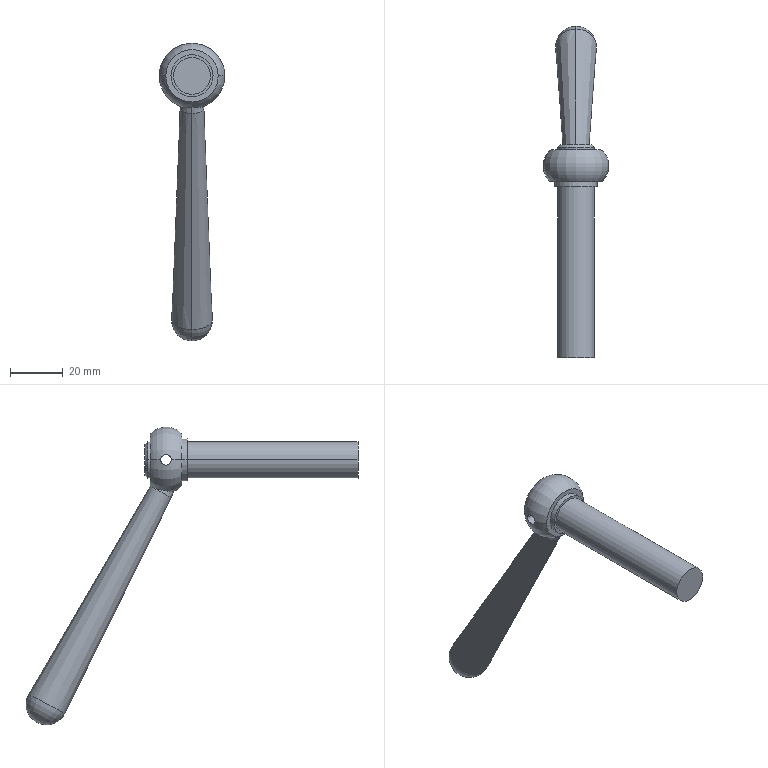Component | SolidWorks | Handle-1 | 1 solid | 23 faces | volume 27831 mm3 | cylinder 8 | cone 6 | plane 5 | torus 4 | commonest cylinder face diameters 14 x4 4 x2 16 x2
STEP:
#1=CARTESIAN_POINT('',(-2.717,8.526,-2.461));
#2=VERTEX_POINT('',#1);
#3=CARTESIAN_POINT('',(-3.189,8.526,-2.461));
#4=VERTEX_POINT('',#3);
#5=CARTESIAN_POINT('',(-2.953,8.526,-2.461));
#6=DIRECTION('',(0.,1.,0.));
#7=DIRECTION('',(1.,0.,0.));
#8=AXIS2_PLACEMENT_3D('',#5,#6,#7);
#9=CIRCLE('',#8,0.2362);
#10=EDGE_CURVE('',#2,#4,#9,.T.);
#11=ORIENTED_EDGE('',*,*,#10,.F.);
#12=CARTESIAN_POINT('',(-2.677,8.487,-2.461));
#13=VERTEX_POINT('',#12);
#14=CARTESIAN_POINT('',(-2.717,8.526,-2.461));
#15=DIRECTION('',(0.7071,-0.7071,-0.));
#16=VECTOR('',#15,39.37);
#17=LINE('',#14,#16);
#18=EDGE_CURVE('',#2,#13,#17,.T.);
#19=ORIENTED_EDGE('',*,*,#18,.T.);
#20=CARTESIAN_POINT('',(-3.228,8.487,-2.461));
#21=VERTEX_POINT('',#20);
#22=CARTESIAN_POINT('',(-2.953,8.487,-2.461));
#23=DIRECTION('',(0.,-1.,0.));
#24=DIRECTION('',(1.,0.,0.));
#25=AXIS2_PLACEMENT_3D('',#22,#23,#24);
#26=CIRCLE('',#25,0.2756);
#27=EDGE_CURVE('',#21,#13,#26,.T.);
#28=ORIENTED_EDGE('',*,*,#27,.F.);
#29=CARTESIAN_POINT('',(-3.189,8.526,-2.461));
#30=DIRECTION('',(-0.7071,-0.7071,0.));
#31=VECTOR('',#30,39.37);
#32=LINE('',#29,#31);
#33=EDGE_CURVE('',#4,#21,#32,.T.);
#34=ORIENTED_EDGE('',*,*,#33,.F.);
#35=EDGE_LOOP('',(#11,#19,#28,#34));
#36=FACE_OUTER_BOUND('',#35,.T.);
#37=CARTESIAN_POINT('',(-2.953,8.526,-2.461));
#38=DIRECTION('',(0.,-1.,0.));
#39=DIRECTION('',(-1.,0.,0.));
#40=AXIS2_PLACEMENT_3D('',#37,#38,#39);
#41=CONICAL_SURFACE('',#40,0.2362,0.7854);
#42=ADVANCED_FACE('',(#36),#41,.T.);
#43=ORIENTED_EDGE('',*,*,#27,.T.);
#44=CARTESIAN_POINT('',(-2.677,8.447,-2.461));
#45=VERTEX_POINT('',#44);
#46=CARTESIAN_POINT('',(-2.677,8.526,-2.461));
#47=DIRECTION('',(0.,-1.,0.));
#48=VECTOR('',#47,39.37);
#49=LINE('',#46,#48);
#50=EDGE_CURVE('',#13,#45,#49,.T.);
#51=ORIENTED_EDGE('',*,*,#50,.T.);
#52=CARTESIAN_POINT('',(-3.228,8.447,-2.461));
#53=VERTEX_POINT('',#52);
#54=CARTESIAN_POINT('',(-2.953,8.447,-2.461));
#55=DIRECTION('',(0.,1.,0.));
#56=DIRECTION('',(1.,0.,0.));
#57=AXIS2_PLACEMENT_3D('',#54,#55,#56);
#58=CIRCLE('',#57,0.2756);
#59=EDGE_CURVE('',#45,#53,#58,.T.);
#60=ORIENTED_EDGE('',*,*,#59,.T.);
#61=CARTESIAN_POINT('',(-3.228,8.526,-2.461));
#62=DIRECTION('',(0.,-1.,0.));
#63=VECTOR('',#62,39.37);
#64=LINE('',#61,#63);
#65=EDGE_CURVE('',#21,#53,#64,.T.);
#66=ORIENTED_EDGE('',*,*,#65,.F.);
#67=EDGE_LOOP('',(#43,#51,#60,#66));
#68=FACE_OUTER_BOUND('',#67,.T.);
#69=CARTESIAN_POINT('',(-2.953,8.526,-2.461));
#70=DIRECTION('',(0.,-1.,0.));
#71=DIRECTION('',(-1.,0.,0.));
#72=AXIS2_PLACEMENT_3D('',#69,#70,#71);
#73=CYLINDRICAL_SURFACE('',#72,0.2756);
#74=ADVANCED_FACE('',(#68),#73,.T.);
#75=CARTESIAN_POINT('',(-3.434,8.29,-2.461));
#76=VERTEX_POINT('',#75);
#77=CARTESIAN_POINT('',(-3.434,8.132,-2.461));
#78=VERTEX_POINT('',#77);
#79=CARTESIAN_POINT('',(-3.434,8.29,-2.461));
#80=CARTESIAN_POINT('',(-3.434,8.29,-2.455));
#81=CARTESIAN_POINT('',(-3.434,8.289,-2.45));
#82=CARTESIAN_POINT('',(-3.434,8.287,-2.44));
#83=CARTESIAN_POINT('',(-3.434,8.286,-2.435));
#84=CARTESIAN_POINT('',(-3.434,8.282,-2.426));
#85=CARTESIAN_POINT('',(-3.435,8.28,-2.421));
#86=CARTESIAN_POINT('',(-3.435,8.274,-2.413));
#87=CARTESIAN_POINT('',(-3.435,8.271,-2.409));
#88=CARTESIAN_POINT('',(-3.436,8.26,-2.398));
#89=CARTESIAN_POINT('',(-3.436,8.251,-2.392));
#90=CARTESIAN_POINT('',(-3.437,8.237,-2.386));
#91=CARTESIAN_POINT('',(-3.437,8.232,-2.384));
#92=CARTESIAN_POINT('',(-3.437,8.222,-2.382));
#93=CARTESIAN_POINT('',(-3.437,8.216,-2.382));
#94=CARTESIAN_POINT('',(-3.437,8.206,-2.382));
#95=CARTESIAN_POINT('',(-3.437,8.201,-2.382));
#96=CARTESIAN_POINT('',(-3.437,8.191,-2.384));
#97=CARTESIAN_POINT('',(-3.437,8.186,-2.386));
#98=CARTESIAN_POINT('',(-3.436,8.172,-2.392));
#99=CARTESIAN_POINT('',(-3.436,8.163,-2.398));
#100=CARTESIAN_POINT('',(-3.435,8.152,-2.409));
#101=CARTESIAN_POINT('',(-3.435,8.149,-2.413));
#102=CARTESIAN_POINT('',(-3.435,8.143,-2.421));
#103=CARTESIAN_POINT('',(-3.434,8.14,-2.426));
#104=CARTESIAN_POINT('',(-3.434,8.136,-2.435));
#105=CARTESIAN_POINT('',(-3.434,8.135,-2.44));
#106=CARTESIAN_POINT('',(-3.434,8.133,-2.45));
#107=CARTESIAN_POINT('',(-3.434,8.132,-2.455));
#108=CARTESIAN_POINT('',(-3.434,8.132,-2.461));
#109=B_SPLINE_CURVE_WITH_KNOTS('',3,(#79,#80,#81,#82,#83,#84,#85,#86,#87,#88,#89,#90,#91,#92,#93,#94,#95,#96,#97,#98,#99,#100,#101,#102,#103,#104,#105,#106,#107,#108),.UNSPECIFIED.,.F.,.F.,(4,2,2,2,2,2,2,2,2,2,2,2,2,2,4),(0.007793,0.008184,0.008575,0.008965,0.009356,0.01014,0.01053,0.01092,0.01131,0.0117,0.01248,0.01287,0.01326,0.01365,0.01405),.UNSPECIFIED.);
#110=EDGE_CURVE('',#76,#78,#109,.T.);
#111=ORIENTED_EDGE('',*,*,#110,.F.);
#112=CARTESIAN_POINT('',(-2.472,8.29,-2.461));
#113=VERTEX_POINT('',#112);
#114=CARTESIAN_POINT('',(-3.613,8.29,-2.461));
#115=DIRECTION('',(1.,0.,0.));
#116=VECTOR('',#115,39.37);
#117=LINE('',#114,#116);
#118=EDGE_CURVE('',#76,#113,#117,.T.);
#119=ORIENTED_EDGE('',*,*,#118,.T.);
#120=CARTESIAN_POINT('',(-2.472,8.132,-2.461));
#121=VERTEX_POINT('',#120);
#122=CARTESIAN_POINT('',(-2.472,8.132,-2.461));
#123=CARTESIAN_POINT('',(-2.472,8.132,-2.45));
#124=CARTESIAN_POINT('',(-2.471,8.135,-2.44));
#125=CARTESIAN_POINT('',(-2.471,8.142,-2.421));
#126=CARTESIAN_POINT('',(-2.471,8.148,-2.412));
#127=CARTESIAN_POINT('',(-2.47,8.159,-2.401));
#128=CARTESIAN_POINT('',(-2.47,8.163,-2.398));
#129=CARTESIAN_POINT('',(-2.469,8.172,-2.392));
#130=CARTESIAN_POINT('',(-2.469,8.176,-2.39));
#131=CARTESIAN_POINT('',(-2.469,8.186,-2.386));
#132=CARTESIAN_POINT('',(-2.469,8.191,-2.384));
#133=CARTESIAN_POINT('',(-2.469,8.201,-2.382));
#134=CARTESIAN_POINT('',(-2.469,8.206,-2.382));
#135=CARTESIAN_POINT('',(-2.469,8.222,-2.382));
#136=CARTESIAN_POINT('',(-2.469,8.232,-2.384));
#137=CARTESIAN_POINT('',(-2.469,8.246,-2.39));
#138=CARTESIAN_POINT('',(-2.469,8.251,-2.392));
#139=CARTESIAN_POINT('',(-2.47,8.259,-2.398));
#140=CARTESIAN_POINT('',(-2.47,8.263,-2.401));
#141=CARTESIAN_POINT('',(-2.47,8.271,-2.409));
#142=CARTESIAN_POINT('',(-2.471,8.274,-2.413));
#143=CARTESIAN_POINT('',(-2.471,8.28,-2.421));
#144=CARTESIAN_POINT('',(-2.471,8.282,-2.426));
#145=CARTESIAN_POINT('',(-2.471,8.286,-2.435));
#146=CARTESIAN_POINT('',(-2.471,8.287,-2.44));
#147=CARTESIAN_POINT('',(-2.472,8.289,-2.45));
#148=CARTESIAN_POINT('',(-2.472,8.29,-2.455));
#149=CARTESIAN_POINT('',(-2.472,8.29,-2.461));
#150=B_SPLINE_CURVE_WITH_KNOTS('',3,(#122,#123,#124,#125,#126,#127,#128,#129,#130,#131,#132,#133,#134,#135,#136,#137,#138,#139,#140,#141,#142,#143,#144,#145,#146,#147,#148,#149),.UNSPECIFIED.,.F.,.F.,(4,2,2,2,2,2,2,2,2,2,2,2,2,4),(0.01097,0.01176,0.01254,0.01293,0.01332,0.01371,0.0141,0.01488,0.01527,0.01566,0.01606,0.01645,0.01684,0.01723),.UNSPECIFIED.);
#151=EDGE_CURVE('',#121,#113,#150,.T.);
#152=ORIENTED_EDGE('',*,*,#151,.F.);
#153=CARTESIAN_POINT('',(-3.613,8.132,-2.461));
#154=DIRECTION('',(1.,0.,0.));
#155=VECTOR('',#154,39.37);
#156=LINE('',#153,#155);
#157=EDGE_CURVE('',#78,#121,#156,.T.);
#158=ORIENTED_EDGE('',*,*,#157,.F.);
#159=EDGE_LOOP('',(#111,#119,#152,#158));
#160=FACE_OUTER_BOUND('',#159,.T.);
#161=CARTESIAN_POINT('',(-3.613,8.211,-2.461));
#162=DIRECTION('',(1.,0.,0.));
#163=DIRECTION('',(0.,-1.,0.));
#164=AXIS2_PLACEMENT_3D('',#161,#162,#163);
#165=CYLINDRICAL_SURFACE('',#164,0.07874);
#166=ADVANCED_FACE('',(#160),#165,.F.);
#167=CARTESIAN_POINT('',(-2.953,10.146,-6.391));
#168=VERTEX_POINT('',#167);
#169=CARTESIAN_POINT('',(-2.953,9.726,-6.258));
#170=VERTEX_POINT('',#169);
#171=CARTESIAN_POINT('',(-2.953,10.,-6.123));
#172=DIRECTION('',(-1.,0.,0.));
#173=DIRECTION('',(0.,0.,1.));
#174=AXIS2_PLACEMENT_3D('',#171,#172,#173);
#175=CIRCLE('',#174,0.305);
#176=EDGE_CURVE('',#168,#170,#175,.T.);
#177=ORIENTED_EDGE('',*,*,#176,.F.);
#178=CARTESIAN_POINT('',(-2.953,10.266,-5.967));
#179=VERTEX_POINT('',#178);
#180=CARTESIAN_POINT('',(-2.953,10.003,-6.121));
#181=DIRECTION('',(1.,-0.,-0.));
#182=DIRECTION('',(0.,1.,0.));
#183=AXIS2_PLACEMENT_3D('',#180,#181,#182);
#184=CIRCLE('',#183,0.305);
#185=EDGE_CURVE('',#168,#179,#184,.T.);
#186=ORIENTED_EDGE('',*,*,#185,.T.);
#187=CARTESIAN_POINT('',(-2.953,9.996,-6.113));
#188=DIRECTION('',(0.,-0.4737,0.8807));
#189=DIRECTION('',(0.,-0.8807,-0.4737));
#190=AXIS2_PLACEMENT_3D('',#187,#188,#189);
#191=CIRCLE('',#190,0.3066);
#192=EDGE_CURVE('',#170,#179,#191,.T.);
#193=ORIENTED_EDGE('',*,*,#192,.F.);
#194=EDGE_LOOP('',(#177,#186,#193));
#195=FACE_OUTER_BOUND('',#194,.T.);
#196=CARTESIAN_POINT('',(-2.953,10.002,-6.122));
#197=DIRECTION('',(0.,-0.4737,0.8807));
#198=DIRECTION('',(0.,-0.8807,-0.4737));
#199=AXIS2_PLACEMENT_3D('',#196,#197,#198);
#200=TOROIDAL_SURFACE('',#199,0.001727,0.305);
#201=ADVANCED_FACE('',(#195),#200,.T.);
#202=CARTESIAN_POINT('',(-2.953,8.131,-3.023));
#203=VERTEX_POINT('',#202);
#204=CARTESIAN_POINT('',(-2.953,8.447,-2.853));
#205=VERTEX_POINT('',#204);
#206=CARTESIAN_POINT('',(-2.953,8.289,-2.938));
#207=DIRECTION('',(0.,-0.4737,0.8807));
#208=DIRECTION('',(0.,-0.8807,-0.4737));
#209=AXIS2_PLACEMENT_3D('',#206,#207,#208);
#210=CIRCLE('',#209,0.1796);
#211=EDGE_CURVE('',#203,#205,#210,.T.);
#212=ORIENTED_EDGE('',*,*,#211,.F.);
#213=CARTESIAN_POINT('',(-2.953,9.726,-6.258));
#214=DIRECTION('',(0.,0.4423,-0.8968));
#215=VECTOR('',#214,39.37);
#216=LINE('',#213,#215);
#217=EDGE_CURVE('',#203,#170,#216,.T.);
#218=ORIENTED_EDGE('',*,*,#217,.T.);
#219=ORIENTED_EDGE('',*,*,#192,.T.);
#220=CARTESIAN_POINT('',(-2.953,10.266,-5.967));
#221=DIRECTION('',(0.,0.5044,-0.8635));
#222=VECTOR('',#221,39.37);
#223=LINE('',#220,#222);
#224=EDGE_CURVE('',#205,#179,#223,.T.);
#225=ORIENTED_EDGE('',*,*,#224,.F.);
#226=EDGE_LOOP('',(#212,#218,#219,#225));
#227=FACE_OUTER_BOUND('',#226,.T.);
#228=CARTESIAN_POINT('',(-2.953,9.996,-6.113));
#229=DIRECTION('',(0.,0.4737,-0.8807));
#230=DIRECTION('',(0.,0.8807,0.4737));
#231=AXIS2_PLACEMENT_3D('',#228,#229,#230);
#232=CONICAL_SURFACE('',#231,0.3066,0.03523);
#233=ADVANCED_FACE('',(#227),#232,.T.);
#234=CARTESIAN_POINT('',(-2.953,8.099,-2.932));
#235=VERTEX_POINT('',#234);
#236=CARTESIAN_POINT('',(-2.953,8.099,-2.932));
#237=CARTESIAN_POINT('',(-2.941,8.099,-2.932));
#238=CARTESIAN_POINT('',(-2.93,8.1,-2.932));
#239=CARTESIAN_POINT('',(-2.907,8.106,-2.932));
#240=CARTESIAN_POINT('',(-2.896,8.109,-2.932));
#241=CARTESIAN_POINT('',(-2.875,8.119,-2.932));
#242=CARTESIAN_POINT('',(-2.865,8.125,-2.932));
#243=CARTESIAN_POINT('',(-2.846,8.139,-2.931));
#244=CARTESIAN_POINT('',(-2.837,8.146,-2.931));
#245=CARTESIAN_POINT('',(-2.821,8.163,-2.93));
#246=CARTESIAN_POINT('',(-2.814,8.173,-2.929));
#247=CARTESIAN_POINT('',(-2.802,8.192,-2.927));
#248=CARTESIAN_POINT('',(-2.796,8.202,-2.926));
#249=CARTESIAN_POINT('',(-2.788,8.224,-2.922));
#250=CARTESIAN_POINT('',(-2.784,8.235,-2.921));
#251=CARTESIAN_POINT('',(-2.779,8.257,-2.916));
#252=CARTESIAN_POINT('',(-2.778,8.268,-2.914));
#253=CARTESIAN_POINT('',(-2.778,8.291,-2.909));
#254=CARTESIAN_POINT('',(-2.778,8.302,-2.906));
#255=CARTESIAN_POINT('',(-2.782,8.324,-2.9));
#256=CARTESIAN_POINT('',(-2.786,8.335,-2.897));
#257=CARTESIAN_POINT('',(-2.794,8.355,-2.89));
#258=CARTESIAN_POINT('',(-2.799,8.365,-2.887));
#259=CARTESIAN_POINT('',(-2.812,8.384,-2.88));
#260=CARTESIAN_POINT('',(-2.819,8.392,-2.877));
#261=CARTESIAN_POINT('',(-2.836,8.408,-2.871));
#262=CARTESIAN_POINT('',(-2.845,8.414,-2.868));
#263=CARTESIAN_POINT('',(-2.864,8.426,-2.863));
#264=CARTESIAN_POINT('',(-2.874,8.431,-2.861));
#265=CARTESIAN_POINT('',(-2.896,8.439,-2.857));
#266=CARTESIAN_POINT('',(-2.907,8.442,-2.856));
#267=CARTESIAN_POINT('',(-2.93,8.446,-2.854));
#268=CARTESIAN_POINT('',(-2.941,8.447,-2.853));
#269=CARTESIAN_POINT('',(-2.953,8.447,-2.853));
#270=B_SPLINE_CURVE_WITH_KNOTS('',3,(#236,#237,#238,#239,#240,#241,#242,#243,#244,#245,#246,#247,#248,#249,#250,#251,#252,#253,#254,#255,#256,#257,#258,#259,#260,#261,#262,#263,#264,#265,#266,#267,#268,#269),.UNSPECIFIED.,.F.,.F.,(4,2,2,2,2,2,2,2,2,2,2,2,2,2,2,2,4),(0.003343,0.004223,0.005103,0.005984,0.006864,0.007744,0.008624,0.009504,0.01038,0.01126,0.01214,0.01302,0.0139,0.01478,0.01566,0.01654,0.01742),.UNSPECIFIED.);
#271=EDGE_CURVE('',#235,#205,#270,.T.);
#272=ORIENTED_EDGE('',*,*,#271,.F.);
#273=CARTESIAN_POINT('',(-2.953,8.131,-3.023));
#274=DIRECTION('',(0.,0.3301,-0.944));
#275=VECTOR('',#274,39.37);
#276=LINE('',#273,#275);
#277=EDGE_CURVE('',#235,#203,#276,.T.);
#278=ORIENTED_EDGE('',*,*,#277,.T.);
#279=ORIENTED_EDGE('',*,*,#211,.T.);
#280=EDGE_LOOP('',(#272,#278,#279));
#281=FACE_OUTER_BOUND('',#280,.T.);
#282=CARTESIAN_POINT('',(-2.953,8.289,-2.938));
#283=DIRECTION('',(0.,0.4737,-0.8807));
#284=DIRECTION('',(0.,0.8807,0.4737));
#285=AXIS2_PLACEMENT_3D('',#282,#283,#284);
#286=CONICAL_SURFACE('',#285,0.1796,0.1571);
#287=ADVANCED_FACE('',(#281),#286,.T.);
#288=CARTESIAN_POINT('',(-2.638,7.975,-2.461));
#289=VERTEX_POINT('',#288);
#290=CARTESIAN_POINT('',(-3.268,7.975,-2.461));
#291=VERTEX_POINT('',#290);
#292=CARTESIAN_POINT('',(-2.953,7.975,-2.461));
#293=DIRECTION('',(0.,1.,0.));
#294=DIRECTION('',(1.,0.,0.));
#295=AXIS2_PLACEMENT_3D('',#292,#293,#294);
#296=CIRCLE('',#295,0.315);
#297=EDGE_CURVE('',#289,#291,#296,.T.);
#298=ORIENTED_EDGE('',*,*,#297,.F.);
#299=CARTESIAN_POINT('',(-2.638,7.896,-2.461));
#300=VERTEX_POINT('',#299);
#301=CARTESIAN_POINT('',(-2.638,7.975,-2.461));
#302=DIRECTION('',(0.,-1.,0.));
#303=VECTOR('',#302,39.37);
#304=LINE('',#301,#303);
#305=EDGE_CURVE('',#289,#300,#304,.T.);
#306=ORIENTED_EDGE('',*,*,#305,.T.);
#307=CARTESIAN_POINT('',(-3.268,7.896,-2.461));
#308=VERTEX_POINT('',#307);
#309=CARTESIAN_POINT('',(-2.953,7.896,-2.461));
#310=DIRECTION('',(0.,1.,0.));
#311=DIRECTION('',(1.,0.,0.));
#312=AXIS2_PLACEMENT_3D('',#309,#310,#311);
#313=CIRCLE('',#312,0.315);
#314=EDGE_CURVE('',#300,#308,#313,.T.);
#315=ORIENTED_EDGE('',*,*,#314,.T.);
#316=CARTESIAN_POINT('',(-3.268,7.975,-2.461));
#317=DIRECTION('',(0.,-1.,0.));
#318=VECTOR('',#317,39.37);
#319=LINE('',#316,#318);
#320=EDGE_CURVE('',#291,#308,#319,.T.);
#321=ORIENTED_EDGE('',*,*,#320,.F.);
#322=EDGE_LOOP('',(#298,#306,#315,#321));
#323=FACE_OUTER_BOUND('',#322,.T.);
#324=CARTESIAN_POINT('',(-2.953,7.975,-2.461));
#325=DIRECTION('',(0.,-1.,0.));
#326=DIRECTION('',(-1.,0.,0.));
#327=AXIS2_PLACEMENT_3D('',#324,#325,#326);
#328=CYLINDRICAL_SURFACE('',#327,0.315);
#329=ADVANCED_FACE('',(#323),#328,.T.);
#330=CARTESIAN_POINT('',(-2.677,5.337,-2.461));
#331=VERTEX_POINT('',#330);
#332=CARTESIAN_POINT('',(-3.228,5.337,-2.461));
#333=VERTEX_POINT('',#332);
#334=CARTESIAN_POINT('',(-2.953,5.337,-2.461));
#335=DIRECTION('',(0.,1.,0.));
#336=DIRECTION('',(1.,0.,0.));
#337=AXIS2_PLACEMENT_3D('',#334,#335,#336);
#338=CIRCLE('',#337,0.2756);
#339=EDGE_CURVE('',#331,#333,#338,.T.);
#340=ORIENTED_EDGE('',*,*,#339,.T.);
#341=CARTESIAN_POINT('',(-3.228,7.896,-2.461));
#342=VERTEX_POINT('',#341);
#343=CARTESIAN_POINT('',(-3.228,5.337,-2.461));
#344=DIRECTION('',(0.,1.,0.));
#345=VECTOR('',#344,39.37);
#346=LINE('',#343,#345);
#347=EDGE_CURVE('',#333,#342,#346,.T.);
#348=ORIENTED_EDGE('',*,*,#347,.T.);
#349=CARTESIAN_POINT('',(-2.677,7.896,-2.461));
#350=VERTEX_POINT('',#349);
#351=CARTESIAN_POINT('',(-2.953,7.896,-2.461));
#352=DIRECTION('',(0.,1.,0.));
#353=DIRECTION('',(1.,0.,0.));
#354=AXIS2_PLACEMENT_3D('',#351,#352,#353);
#355=CIRCLE('',#354,0.2756);
#356=EDGE_CURVE('',#350,#342,#355,.T.);
#357=ORIENTED_EDGE('',*,*,#356,.F.);
#358=CARTESIAN_POINT('',(-2.677,5.337,-2.461));
#359=DIRECTION('',(0.,1.,0.));
#360=VECTOR('',#359,39.37);
#361=LINE('',#358,#360);
#362=EDGE_CURVE('',#331,#350,#361,.T.);
#363=ORIENTED_EDGE('',*,*,#362,.F.);
#364=EDGE_LOOP('',(#340,#348,#357,#363));
#365=FACE_OUTER_BOUND('',#364,.T.);
#366=CARTESIAN_POINT('',(-2.953,5.337,-2.461));
#367=DIRECTION('',(0.,1.,0.));
#368=DIRECTION('',(1.,0.,0.));
#369=AXIS2_PLACEMENT_3D('',#366,#367,#368);
#370=CYLINDRICAL_SURFACE('',#369,0.2756);
#371=ADVANCED_FACE('',(#365),#370,.T.);
#372=CARTESIAN_POINT('',(-2.56,7.975,-2.461));
#373=VERTEX_POINT('',#372);
#374=CARTESIAN_POINT('',(-3.345,7.975,-2.461));
#375=VERTEX_POINT('',#374);
#376=CARTESIAN_POINT('',(-2.953,7.975,-2.461));
#377=DIRECTION('',(0.,1.,0.));
#378=DIRECTION('',(1.,0.,0.));
#379=AXIS2_PLACEMENT_3D('',#376,#377,#378);
#380=CIRCLE('',#379,0.3927);
#381=EDGE_CURVE('',#373,#375,#380,.T.);
#382=ORIENTED_EDGE('',*,*,#381,.T.);
#383=CARTESIAN_POINT('',(-3.109,8.211,-2.461));
#384=DIRECTION('',(0.,0.,-1.));
#385=DIRECTION('',(-1.,0.,0.));
#386=AXIS2_PLACEMENT_3D('',#383,#384,#385);
#387=CIRCLE('',#386,0.3341);
#388=EDGE_CURVE('',#375,#78,#387,.T.);
#389=ORIENTED_EDGE('',*,*,#388,.T.);
#390=CARTESIAN_POINT('',(-3.434,8.132,-2.461));
#391=CARTESIAN_POINT('',(-3.434,8.132,-2.466));
#392=CARTESIAN_POINT('',(-3.434,8.133,-2.471));
#393=CARTESIAN_POINT('',(-3.434,8.135,-2.481));
#394=CARTESIAN_POINT('',(-3.434,8.136,-2.486));
#395=CARTESIAN_POINT('',(-3.435,8.142,-2.5));
#396=CARTESIAN_POINT('',(-3.435,8.148,-2.509));
#397=CARTESIAN_POINT('',(-3.436,8.159,-2.52));
#398=CARTESIAN_POINT('',(-3.436,8.163,-2.523));
#399=CARTESIAN_POINT('',(-3.436,8.172,-2.529));
#400=CARTESIAN_POINT('',(-3.436,8.176,-2.531));
#401=CARTESIAN_POINT('',(-3.437,8.186,-2.535));
#402=CARTESIAN_POINT('',(-3.437,8.191,-2.537));
#403=CARTESIAN_POINT('',(-3.437,8.201,-2.539));
#404=CARTESIAN_POINT('',(-3.437,8.206,-2.539));
#405=CARTESIAN_POINT('',(-3.437,8.222,-2.539));
#406=CARTESIAN_POINT('',(-3.437,8.232,-2.537));
#407=CARTESIAN_POINT('',(-3.436,8.246,-2.531));
#408=CARTESIAN_POINT('',(-3.436,8.251,-2.529));
#409=CARTESIAN_POINT('',(-3.436,8.259,-2.523));
#410=CARTESIAN_POINT('',(-3.436,8.263,-2.52));
#411=CARTESIAN_POINT('',(-3.435,8.271,-2.513));
#412=CARTESIAN_POINT('',(-3.435,8.274,-2.509));
#413=CARTESIAN_POINT('',(-3.435,8.28,-2.5));
#414=CARTESIAN_POINT('',(-3.434,8.282,-2.495));
#415=CARTESIAN_POINT('',(-3.434,8.288,-2.481));
#416=CARTESIAN_POINT('',(-3.434,8.29,-2.471));
#417=CARTESIAN_POINT('',(-3.434,8.29,-2.461));
#418=B_SPLINE_CURVE_WITH_KNOTS('',3,(#390,#391,#392,#393,#394,#395,#396,#397,#398,#399,#400,#401,#402,#403,#404,#405,#406,#407,#408,#409,#410,#411,#412,#413,#414,#415,#416,#417),.UNSPECIFIED.,.F.,.F.,(4,2,2,2,2,2,2,2,2,2,2,2,2,4),(0.001536,0.001927,0.002318,0.003101,0.003492,0.003883,0.004274,0.004665,0.005447,0.005838,0.006229,0.00662,0.007011,0.007793),.UNSPECIFIED.);
#419=EDGE_CURVE('',#78,#76,#418,.T.);
#420=ORIENTED_EDGE('',*,*,#419,.T.);
#421=CARTESIAN_POINT('',(-3.345,8.447,-2.461));
#422=VERTEX_POINT('',#421);
#423=CARTESIAN_POINT('',(-3.109,8.211,-2.461));
#424=DIRECTION('',(0.,0.,-1.));
#425=DIRECTION('',(-1.,0.,0.));
#426=AXIS2_PLACEMENT_3D('',#423,#424,#425);
#427=CIRCLE('',#426,0.3341);
#428=EDGE_CURVE('',#76,#422,#427,.T.);
#429=ORIENTED_EDGE('',*,*,#428,.T.);
#430=CARTESIAN_POINT('',(-2.953,8.447,-2.461));
#431=DIRECTION('',(0.,1.,0.));
#432=DIRECTION('',(1.,0.,0.));
#433=AXIS2_PLACEMENT_3D('',#430,#431,#432);
#434=CIRCLE('',#433,0.3927);
#435=EDGE_CURVE('',#205,#422,#434,.T.);
#436=ORIENTED_EDGE('',*,*,#435,.F.);
#437=CARTESIAN_POINT('',(-2.953,8.447,-2.853));
#438=CARTESIAN_POINT('',(-2.964,8.447,-2.853));
#439=CARTESIAN_POINT('',(-2.976,8.446,-2.854));
#440=CARTESIAN_POINT('',(-2.999,8.442,-2.856));
#441=CARTESIAN_POINT('',(-3.01,8.439,-2.857));
#442=CARTESIAN_POINT('',(-3.031,8.431,-2.861));
#443=CARTESIAN_POINT('',(-3.042,8.426,-2.863));
#444=CARTESIAN_POINT('',(-3.061,8.414,-2.868));
#445=CARTESIAN_POINT('',(-3.07,8.408,-2.871));
#446=CARTESIAN_POINT('',(-3.086,8.392,-2.877));
#447=CARTESIAN_POINT('',(-3.093,8.384,-2.88));
#448=CARTESIAN_POINT('',(-3.106,8.365,-2.887));
#449=CARTESIAN_POINT('',(-3.111,8.355,-2.89));
#450=CARTESIAN_POINT('',(-3.12,8.335,-2.897));
#451=CARTESIAN_POINT('',(-3.123,8.324,-2.9));
#452=CARTESIAN_POINT('',(-3.127,8.302,-2.906));
#453=CARTESIAN_POINT('',(-3.128,8.291,-2.909));
#454=CARTESIAN_POINT('',(-3.128,8.268,-2.914));
#455=CARTESIAN_POINT('',(-3.126,8.257,-2.916));
#456=CARTESIAN_POINT('',(-3.121,8.234,-2.921));
#457=CARTESIAN_POINT('',(-3.118,8.223,-2.922));
#458=CARTESIAN_POINT('',(-3.109,8.202,-2.926));
#459=CARTESIAN_POINT('',(-3.104,8.192,-2.927));
#460=CARTESIAN_POINT('',(-3.091,8.172,-2.929));
#461=CARTESIAN_POINT('',(-3.084,8.163,-2.93));
#462=CARTESIAN_POINT('',(-3.068,8.146,-2.931));
#463=CARTESIAN_POINT('',(-3.059,8.139,-2.931));
#464=CARTESIAN_POINT('',(-3.041,8.125,-2.932));
#465=CARTESIAN_POINT('',(-3.031,8.119,-2.932));
#466=CARTESIAN_POINT('',(-3.01,8.109,-2.932));
#467=CARTESIAN_POINT('',(-2.999,8.106,-2.932));
#468=CARTESIAN_POINT('',(-2.976,8.1,-2.932));
#469=CARTESIAN_POINT('',(-2.964,8.099,-2.932));
#470=CARTESIAN_POINT('',(-2.953,8.099,-2.932));
#471=B_SPLINE_CURVE_WITH_KNOTS('',3,(#437,#438,#439,#440,#441,#442,#443,#444,#445,#446,#447,#448,#449,#450,#451,#452,#453,#454,#455,#456,#457,#458,#459,#460,#461,#462,#463,#464,#465,#466,#467,#468,#469,#470),.UNSPECIFIED.,.F.,.F.,(4,2,2,2,2,2,2,2,2,2,2,2,2,2,2,2,4),(0.01742,0.0183,0.01918,0.02006,0.02094,0.02182,0.0227,0.02358,0.02446,0.02534,0.02622,0.0271,0.02798,0.02886,0.02974,0.03062,0.0315),.UNSPECIFIED.);
#472=EDGE_CURVE('',#205,#235,#471,.T.);
#473=ORIENTED_EDGE('',*,*,#472,.T.);
#474=ORIENTED_EDGE('',*,*,#271,.T.);
#475=CARTESIAN_POINT('',(-2.56,8.447,-2.461));
#476=VERTEX_POINT('',#475);
#477=CARTESIAN_POINT('',(-2.953,8.447,-2.461));
#478=DIRECTION('',(0.,1.,0.));
#479=DIRECTION('',(1.,0.,0.));
#480=AXIS2_PLACEMENT_3D('',#477,#478,#479);
#481=CIRCLE('',#480,0.3927);
#482=EDGE_CURVE('',#476,#205,#481,.T.);
#483=ORIENTED_EDGE('',*,*,#482,.F.);
#484=CARTESIAN_POINT('',(-2.796,8.211,-2.461));
#485=DIRECTION('',(0.,0.,1.));
#486=DIRECTION('',(1.,0.,0.));
#487=AXIS2_PLACEMENT_3D('',#484,#485,#486);
#488=CIRCLE('',#487,0.3341);
#489=EDGE_CURVE('',#113,#476,#488,.T.);
#490=ORIENTED_EDGE('',*,*,#489,.F.);
#491=CARTESIAN_POINT('',(-2.472,8.29,-2.461));
#492=CARTESIAN_POINT('',(-2.472,8.29,-2.466));
#493=CARTESIAN_POINT('',(-2.472,8.289,-2.471));
#494=CARTESIAN_POINT('',(-2.471,8.287,-2.481));
#495=CARTESIAN_POINT('',(-2.471,8.286,-2.486));
#496=CARTESIAN_POINT('',(-2.471,8.282,-2.496));
#497=CARTESIAN_POINT('',(-2.471,8.28,-2.5));
#498=CARTESIAN_POINT('',(-2.471,8.274,-2.509));
#499=CARTESIAN_POINT('',(-2.47,8.271,-2.513));
#500=CARTESIAN_POINT('',(-2.47,8.26,-2.524));
#501=CARTESIAN_POINT('',(-2.469,8.251,-2.529));
#502=CARTESIAN_POINT('',(-2.469,8.237,-2.535));
#503=CARTESIAN_POINT('',(-2.469,8.232,-2.537));
#504=CARTESIAN_POINT('',(-2.469,8.221,-2.539));
#505=CARTESIAN_POINT('',(-2.469,8.216,-2.539));
#506=CARTESIAN_POINT('',(-2.469,8.206,-2.539));
#507=CARTESIAN_POINT('',(-2.469,8.201,-2.539));
#508=CARTESIAN_POINT('',(-2.469,8.191,-2.537));
#509=CARTESIAN_POINT('',(-2.469,8.186,-2.535));
#510=CARTESIAN_POINT('',(-2.469,8.176,-2.531));
#511=CARTESIAN_POINT('',(-2.469,8.172,-2.529));
#512=CARTESIAN_POINT('',(-2.47,8.163,-2.523));
#513=CARTESIAN_POINT('',(-2.47,8.159,-2.52));
#514=CARTESIAN_POINT('',(-2.47,8.152,-2.513));
#515=CARTESIAN_POINT('',(-2.471,8.149,-2.509));
#516=CARTESIAN_POINT('',(-2.471,8.143,-2.5));
#517=CARTESIAN_POINT('',(-2.471,8.14,-2.496));
#518=CARTESIAN_POINT('',(-2.471,8.136,-2.486));
#519=CARTESIAN_POINT('',(-2.471,8.135,-2.481));
#520=CARTESIAN_POINT('',(-2.472,8.133,-2.471));
#521=CARTESIAN_POINT('',(-2.472,8.132,-2.466));
#522=CARTESIAN_POINT('',(-2.472,8.132,-2.461));
#523=B_SPLINE_CURVE_WITH_KNOTS('',3,(#491,#492,#493,#494,#495,#496,#497,#498,#499,#500,#501,#502,#503,#504,#505,#506,#507,#508,#509,#510,#511,#512,#513,#514,#515,#516,#517,#518,#519,#520,#521,#522),.UNSPECIFIED.,.F.,.F.,(4,2,2,2,2,2,2,2,2,2,2,2,2,2,2,4),(0.004719,0.00511,0.005501,0.005892,0.006283,0.007065,0.007456,0.007846,0.008237,0.008628,0.009019,0.00941,0.009801,0.01019,0.01058,0.01097),.UNSPECIFIED.);
#524=EDGE_CURVE('',#113,#121,#523,.T.);
#525=ORIENTED_EDGE('',*,*,#524,.T.);
#526=CARTESIAN_POINT('',(-2.796,8.211,-2.461));
#527=DIRECTION('',(0.,0.,1.));
#528=DIRECTION('',(1.,0.,0.));
#529=AXIS2_PLACEMENT_3D('',#526,#527,#528);
#530=CIRCLE('',#529,0.3341);
#531=EDGE_CURVE('',#373,#121,#530,.T.);
#532=ORIENTED_EDGE('',*,*,#531,.F.);
#533=EDGE_LOOP('',(#382,#389,#420,#429,#436,#473,#474,#483,#490,#525,#532));
#534=FACE_OUTER_BOUND('',#533,.T.);
#535=CARTESIAN_POINT('',(-2.953,8.211,-2.461));
#536=DIRECTION('',(0.,1.,0.));
#537=DIRECTION('',(1.,0.,0.));
#538=AXIS2_PLACEMENT_3D('',#535,#536,#537);
#539=TOROIDAL_SURFACE('',#538,0.1564,0.3341);
#540=ADVANCED_FACE('',(#534),#539,.T.);
#541=ORIENTED_EDGE('',*,*,#388,.F.);
#542=CARTESIAN_POINT('',(-2.953,7.975,-2.461));
#543=DIRECTION('',(0.,1.,0.));
#544=DIRECTION('',(1.,0.,0.));
#545=AXIS2_PLACEMENT_3D('',#542,#543,#544);
#546=CIRCLE('',#545,0.3927);
#547=EDGE_CURVE('',#375,#373,#546,.T.);
#548=ORIENTED_EDGE('',*,*,#547,.T.);
#549=ORIENTED_EDGE('',*,*,#531,.T.);
#550=ORIENTED_EDGE('',*,*,#151,.T.);
#551=ORIENTED_EDGE('',*,*,#489,.T.);
#552=CARTESIAN_POINT('',(-2.953,8.447,-2.461));
#553=DIRECTION('',(0.,1.,0.));
#554=DIRECTION('',(1.,0.,0.));
#555=AXIS2_PLACEMENT_3D('',#552,#553,#554);
#556=CIRCLE('',#555,0.3927);
#557=EDGE_CURVE('',#422,#476,#556,.T.);
#558=ORIENTED_EDGE('',*,*,#557,.F.);
#559=ORIENTED_EDGE('',*,*,#428,.F.);
#560=ORIENTED_EDGE('',*,*,#110,.T.);
#561=EDGE_LOOP('',(#541,#548,#549,#550,#551,#558,#559,#560));
#562=FACE_OUTER_BOUND('',#561,.T.);
#563=CARTESIAN_POINT('',(-2.953,8.211,-2.461));
#564=DIRECTION('',(0.,1.,0.));
#565=DIRECTION('',(1.,0.,0.));
#566=AXIS2_PLACEMENT_3D('',#563,#564,#565);
#567=TOROIDAL_SURFACE('',#566,0.1564,0.3341);
#568=ADVANCED_FACE('',(#562),#567,.T.);
#569=ORIENTED_EDGE('',*,*,#347,.F.);
#570=CARTESIAN_POINT('',(-2.953,5.337,-2.461));
#571=DIRECTION('',(0.,1.,0.));
#572=DIRECTION('',(1.,0.,0.));
#573=AXIS2_PLACEMENT_3D('',#570,#571,#572);
#574=CIRCLE('',#573,0.2756);
#575=EDGE_CURVE('',#333,#331,#574,.T.);
#576=ORIENTED_EDGE('',*,*,#575,.T.);
#577=ORIENTED_EDGE('',*,*,#362,.T.);
#578=CARTESIAN_POINT('',(-2.953,7.896,-2.461));
#579=DIRECTION('',(0.,1.,0.));
#580=DIRECTION('',(1.,0.,0.));
#581=AXIS2_PLACEMENT_3D('',#578,#579,#580);
#582=CIRCLE('',#581,0.2756);
#583=EDGE_CURVE('',#342,#350,#582,.T.);
#584=ORIENTED_EDGE('',*,*,#583,.F.);
#585=EDGE_LOOP('',(#569,#576,#577,#584));
#586=FACE_OUTER_BOUND('',#585,.T.);
#587=CARTESIAN_POINT('',(-2.953,5.337,-2.461));
#588=DIRECTION('',(0.,1.,0.));
#589=DIRECTION('',(1.,0.,0.));
#590=AXIS2_PLACEMENT_3D('',#587,#588,#589);
#591=CYLINDRICAL_SURFACE('',#590,0.2756);
#592=ADVANCED_FACE('',(#586),#591,.T.);
#593=ORIENTED_EDGE('',*,*,#339,.F.);
#594=ORIENTED_EDGE('',*,*,#575,.F.);
#595=EDGE_LOOP('',(#593,#594));
#596=FACE_OUTER_BOUND('',#595,.T.);
#597=CARTESIAN_POINT('',(-2.953,5.337,-2.461));
#598=DIRECTION('',(0.,1.,0.));
#599=DIRECTION('',(1.,0.,0.));
#600=AXIS2_PLACEMENT_3D('',#597,#598,#599);
#601=PLANE('',#600);
#602=ADVANCED_FACE('',(#596),#601,.F.);
#603=ORIENTED_EDGE('',*,*,#305,.F.);
#604=CARTESIAN_POINT('',(-2.953,7.975,-2.461));
#605=DIRECTION('',(0.,1.,0.));
#606=DIRECTION('',(1.,0.,0.));
#607=AXIS2_PLACEMENT_3D('',#604,#605,#606);
#608=CIRCLE('',#607,0.315);
#609=EDGE_CURVE('',#291,#289,#608,.T.);
#610=ORIENTED_EDGE('',*,*,#609,.F.);
#611=ORIENTED_EDGE('',*,*,#320,.T.);
#612=CARTESIAN_POINT('',(-2.953,7.896,-2.461));
#613=DIRECTION('',(0.,1.,0.));
#614=DIRECTION('',(1.,0.,0.));
#615=AXIS2_PLACEMENT_3D('',#612,#613,#614);
#616=CIRCLE('',#615,0.315);
#617=EDGE_CURVE('',#308,#300,#616,.T.);
#618=ORIENTED_EDGE('',*,*,#617,.T.);
#619=EDGE_LOOP('',(#603,#610,#611,#618));
#620=FACE_OUTER_BOUND('',#619,.T.);
#621=CARTESIAN_POINT('',(-2.953,7.975,-2.461));
#622=DIRECTION('',(0.,-1.,0.));
#623=DIRECTION('',(-1.,0.,0.));
#624=AXIS2_PLACEMENT_3D('',#621,#622,#623);
#625=CYLINDRICAL_SURFACE('',#624,0.315);
#626=ADVANCED_FACE('',(#620),#625,.T.);
#627=ORIENTED_EDGE('',*,*,#356,.T.);
#628=ORIENTED_EDGE('',*,*,#583,.T.);
#629=EDGE_LOOP('',(#627,#628));
#630=FACE_BOUND('',#629,.T.);
#631=ORIENTED_EDGE('',*,*,#617,.F.);
#632=ORIENTED_EDGE('',*,*,#314,.F.);
#633=EDGE_LOOP('',(#631,#632));
#634=FACE_OUTER_BOUND('',#633,.T.);
#635=CARTESIAN_POINT('',(-2.953,7.896,-2.461));
#636=DIRECTION('',(0.,1.,0.));
#637=DIRECTION('',(1.,0.,0.));
#638=AXIS2_PLACEMENT_3D('',#635,#636,#637);
#639=PLANE('',#638);
#640=ADVANCED_FACE('',(#630,#634),#639,.F.);
#641=CARTESIAN_POINT('',(-2.953,8.447,-2.461));
#642=DIRECTION('',(0.,1.,0.));
#643=DIRECTION('',(1.,0.,0.));
#644=AXIS2_PLACEMENT_3D('',#641,#642,#643);
#645=CIRCLE('',#644,0.2756);
#646=EDGE_CURVE('',#53,#45,#645,.T.);
#647=ORIENTED_EDGE('',*,*,#646,.F.);
#648=ORIENTED_EDGE('',*,*,#59,.F.);
#649=EDGE_LOOP('',(#647,#648));
#650=FACE_BOUND('',#649,.T.);
#651=ORIENTED_EDGE('',*,*,#435,.T.);
#652=ORIENTED_EDGE('',*,*,#557,.T.);
#653=ORIENTED_EDGE('',*,*,#482,.T.);
#654=EDGE_LOOP('',(#651,#652,#653));
#655=FACE_OUTER_BOUND('',#654,.T.);
#656=CARTESIAN_POINT('',(-2.953,8.447,-2.461));
#657=DIRECTION('',(0.,1.,0.));
#658=DIRECTION('',(1.,0.,0.));
#659=AXIS2_PLACEMENT_3D('',#656,#657,#658);
#660=PLANE('',#659);
#661=ADVANCED_FACE('',(#650,#655),#660,.T.);
#662=ORIENTED_EDGE('',*,*,#609,.T.);
#663=ORIENTED_EDGE('',*,*,#297,.T.);
#664=EDGE_LOOP('',(#662,#663));
#665=FACE_BOUND('',#664,.T.);
#666=ORIENTED_EDGE('',*,*,#381,.F.);
#667=ORIENTED_EDGE('',*,*,#547,.F.);
#668=EDGE_LOOP('',(#666,#667));
#669=FACE_OUTER_BOUND('',#668,.T.);
#670=CARTESIAN_POINT('',(-2.953,7.975,-2.461));
#671=DIRECTION('',(0.,-1.,0.));
#672=DIRECTION('',(-1.,0.,0.));
#673=AXIS2_PLACEMENT_3D('',#670,#671,#672);
#674=PLANE('',#673);
#675=ADVANCED_FACE('',(#665,#669),#674,.T.);
#676=ORIENTED_EDGE('',*,*,#277,.F.);
#677=ORIENTED_EDGE('',*,*,#472,.F.);
#678=CARTESIAN_POINT('',(-2.953,8.289,-2.938));
#679=DIRECTION('',(0.,-0.4737,0.8807));
#680=DIRECTION('',(0.,-0.8807,-0.4737));
#681=AXIS2_PLACEMENT_3D('',#678,#679,#680);
#682=CIRCLE('',#681,0.1796);
#683=EDGE_CURVE('',#205,#203,#682,.T.);
#684=ORIENTED_EDGE('',*,*,#683,.T.);
#685=EDGE_LOOP('',(#676,#677,#684));
#686=FACE_OUTER_BOUND('',#685,.T.);
#687=CARTESIAN_POINT('',(-2.953,8.289,-2.938));
#688=DIRECTION('',(0.,0.4737,-0.8807));
#689=DIRECTION('',(0.,0.8807,0.4737));
#690=AXIS2_PLACEMENT_3D('',#687,#688,#689);
#691=CONICAL_SURFACE('',#690,0.1796,0.1571);
#692=ADVANCED_FACE('',(#686),#691,.T.);
#693=ORIENTED_EDGE('',*,*,#217,.F.);
#694=ORIENTED_EDGE('',*,*,#683,.F.);
#695=ORIENTED_EDGE('',*,*,#224,.T.);
#696=CARTESIAN_POINT('',(-2.953,9.996,-6.113));
#697=DIRECTION('',(0.,-0.4737,0.8807));
#698=DIRECTION('',(0.,-0.8807,-0.4737));
#699=AXIS2_PLACEMENT_3D('',#696,#697,#698);
#700=CIRCLE('',#699,0.3066);
#701=EDGE_CURVE('',#179,#170,#700,.T.);
#702=ORIENTED_EDGE('',*,*,#701,.T.);
#703=EDGE_LOOP('',(#693,#694,#695,#702));
#704=FACE_OUTER_BOUND('',#703,.T.);
#705=CARTESIAN_POINT('',(-2.953,9.996,-6.113));
#706=DIRECTION('',(0.,0.4737,-0.8807));
#707=DIRECTION('',(0.,0.8807,0.4737));
#708=AXIS2_PLACEMENT_3D('',#705,#706,#707);
#709=CONICAL_SURFACE('',#708,0.3066,0.03523);
#710=ADVANCED_FACE('',(#704),#709,.T.);
#711=ORIENTED_EDGE('',*,*,#185,.F.);
#712=ORIENTED_EDGE('',*,*,#176,.T.);
#713=ORIENTED_EDGE('',*,*,#701,.F.);
#714=EDGE_LOOP('',(#711,#712,#713));
#715=FACE_OUTER_BOUND('',#714,.T.);
#716=CARTESIAN_POINT('',(-2.953,10.002,-6.122));
#717=DIRECTION('',(0.,-0.4737,0.8807));
#718=DIRECTION('',(0.,-0.8807,-0.4737));
#719=AXIS2_PLACEMENT_3D('',#716,#717,#718);
#720=TOROIDAL_SURFACE('',#719,0.001727,0.305);
#721=ADVANCED_FACE('',(#715),#720,.T.);
#722=ORIENTED_EDGE('',*,*,#118,.F.);
#723=ORIENTED_EDGE('',*,*,#419,.F.);
#724=ORIENTED_EDGE('',*,*,#157,.T.);
#725=ORIENTED_EDGE('',*,*,#524,.F.);
#726=EDGE_LOOP('',(#722,#723,#724,#725));
#727=FACE_OUTER_BOUND('',#726,.T.);
#728=CARTESIAN_POINT('',(-3.613,8.211,-2.461));
#729=DIRECTION('',(1.,0.,0.));
#730=DIRECTION('',(0.,-1.,0.));
#731=AXIS2_PLACEMENT_3D('',#728,#729,#730);
#732=CYLINDRICAL_SURFACE('',#731,0.07874);
#733=ADVANCED_FACE('',(#727),#732,.F.);
#734=ORIENTED_EDGE('',*,*,#50,.F.);
#735=CARTESIAN_POINT('',(-2.953,8.487,-2.461));
#736=DIRECTION('',(0.,-1.,0.));
#737=DIRECTION('',(1.,0.,0.));
#738=AXIS2_PLACEMENT_3D('',#735,#736,#737);
#739=CIRCLE('',#738,0.2756);
#740=EDGE_CURVE('',#13,#21,#739,.T.);
#741=ORIENTED_EDGE('',*,*,#740,.T.);
#742=ORIENTED_EDGE('',*,*,#65,.T.);
#743=ORIENTED_EDGE('',*,*,#646,.T.);
#744=EDGE_LOOP('',(#734,#741,#742,#743));
#745=FACE_OUTER_BOUND('',#744,.T.);
#746=CARTESIAN_POINT('',(-2.953,8.526,-2.461));
#747=DIRECTION('',(0.,-1.,0.));
#748=DIRECTION('',(-1.,0.,0.));
#749=AXIS2_PLACEMENT_3D('',#746,#747,#748);
#750=CYLINDRICAL_SURFACE('',#749,0.2756);
#751=ADVANCED_FACE('',(#745),#750,.T.);
#752=CARTESIAN_POINT('',(-2.953,8.526,-2.461));
#753=DIRECTION('',(0.,1.,0.));
#754=DIRECTION('',(1.,0.,0.));
#755=AXIS2_PLACEMENT_3D('',#752,#753,#754);
#756=CIRCLE('',#755,0.2362);
#757=EDGE_CURVE('',#4,#2,#756,.T.);
#758=ORIENTED_EDGE('',*,*,#757,.T.);
#759=ORIENTED_EDGE('',*,*,#10,.T.);
#760=EDGE_LOOP('',(#758,#759));
#761=FACE_OUTER_BOUND('',#760,.T.);
#762=CARTESIAN_POINT('',(-2.953,8.526,-2.461));
#763=DIRECTION('',(0.,1.,0.));
#764=DIRECTION('',(1.,0.,0.));
#765=AXIS2_PLACEMENT_3D('',#762,#763,#764);
#766=PLANE('',#765);
#767=ADVANCED_FACE('',(#761),#766,.T.);
#768=ORIENTED_EDGE('',*,*,#18,.F.);
#769=ORIENTED_EDGE('',*,*,#757,.F.);
#770=ORIENTED_EDGE('',*,*,#33,.T.);
#771=ORIENTED_EDGE('',*,*,#740,.F.);
#772=EDGE_LOOP('',(#768,#769,#770,#771));
#773=FACE_OUTER_BOUND('',#772,.T.);
#774=CARTESIAN_POINT('',(-2.953,8.526,-2.461));
#775=DIRECTION('',(0.,-1.,0.));
#776=DIRECTION('',(-1.,0.,0.));
#777=AXIS2_PLACEMENT_3D('',#774,#775,#776);
#778=CONICAL_SURFACE('',#777,0.2362,0.7854);
#779=ADVANCED_FACE('',(#773),#778,.T.);
#780=CLOSED_SHELL('',(#42,#74,#166,#201,#233,#287,#329,#371,#540,#568,#592,#602,#626,#640,#661,#675,#692,#710,#721,#733,#751,#767,#779));
#781=MANIFOLD_SOLID_BREP('',#780);
#782=CARTESIAN_POINT('',(0.,0.,0.));
#783=DIRECTION('',(0.,0.,1.));
#784=DIRECTION('',(1.,0.,0.));
#785=AXIS2_PLACEMENT_3D('',#782,#783,#784);
#786=(LENGTH_UNIT()NAMED_UNIT(*)SI_UNIT($,.METRE.));
#787=LENGTH_MEASURE_WITH_UNIT(LENGTH_MEASURE(0.0254),#786);
#788=DIMENSIONAL_EXPONENTS(1.,0.,0.,0.,0.,0.,0.);
#789=(CONVERSION_BASED_UNIT('',#787)LENGTH_UNIT()NAMED_UNIT(#788));
#790=UNCERTAINTY_MEASURE_WITH_UNIT(LENGTH_MEASURE(0.00001),#789,'','');
#791=(NAMED_UNIT(*)PLANE_ANGLE_UNIT()SI_UNIT($,.RADIAN.));
#792=(NAMED_UNIT(*)SI_UNIT($,.STERADIAN.)SOLID_ANGLE_UNIT());
#793=(GEOMETRIC_REPRESENTATION_CONTEXT(3)GLOBAL_UNCERTAINTY_ASSIGNED_CONTEXT((#790))GLOBAL_UNIT_ASSIGNED_CONTEXT((#789,#791,#792))REPRESENTATION_CONTEXT('',''));
#794=ADVANCED_BREP_SHAPE_REPRESENTATION('',(#781,#785),#793);
#795=COLOUR_RGB('',0.7922,0.8196,0.9333);
#796=FILL_AREA_STYLE_COLOUR('',#795);
#797=FILL_AREA_STYLE('',(#796));
#798=SURFACE_STYLE_FILL_AREA(#797);
#799=SURFACE_SIDE_STYLE('',(#798));
#800=SURFACE_STYLE_USAGE(.BOTH.,#799);
#801=PRESENTATION_STYLE_ASSIGNMENT((#800));
#802=STYLED_ITEM('',(#801),#781);
#803=(LENGTH_UNIT()NAMED_UNIT(*)SI_UNIT($,.METRE.));
#804=LENGTH_MEASURE_WITH_UNIT(LENGTH_MEASURE(0.0254),#803);
#805=DIMENSIONAL_EXPONENTS(1.,0.,0.,0.,0.,0.,0.);
#806=(CONVERSION_BASED_UNIT('',#804)LENGTH_UNIT()NAMED_UNIT(#805));
#807=UNCERTAINTY_MEASURE_WITH_UNIT(LENGTH_MEASURE(0.00001),#806,'','');
#808=(NAMED_UNIT(*)PLANE_ANGLE_UNIT()SI_UNIT($,.RADIAN.));
#809=(NAMED_UNIT(*)SI_UNIT($,.STERADIAN.)SOLID_ANGLE_UNIT());
#810=(GEOMETRIC_REPRESENTATION_CONTEXT(3)GLOBAL_UNCERTAINTY_ASSIGNED_CONTEXT((#807))GLOBAL_UNIT_ASSIGNED_CONTEXT((#806,#808,#809))REPRESENTATION_CONTEXT('',''));
#811=MECHANICAL_DESIGN_GEOMETRIC_PRESENTATION_REPRESENTATION('',(#802),#810);
#812=PRESENTATION_LAYER_ASSIGNMENT('','',(#802));